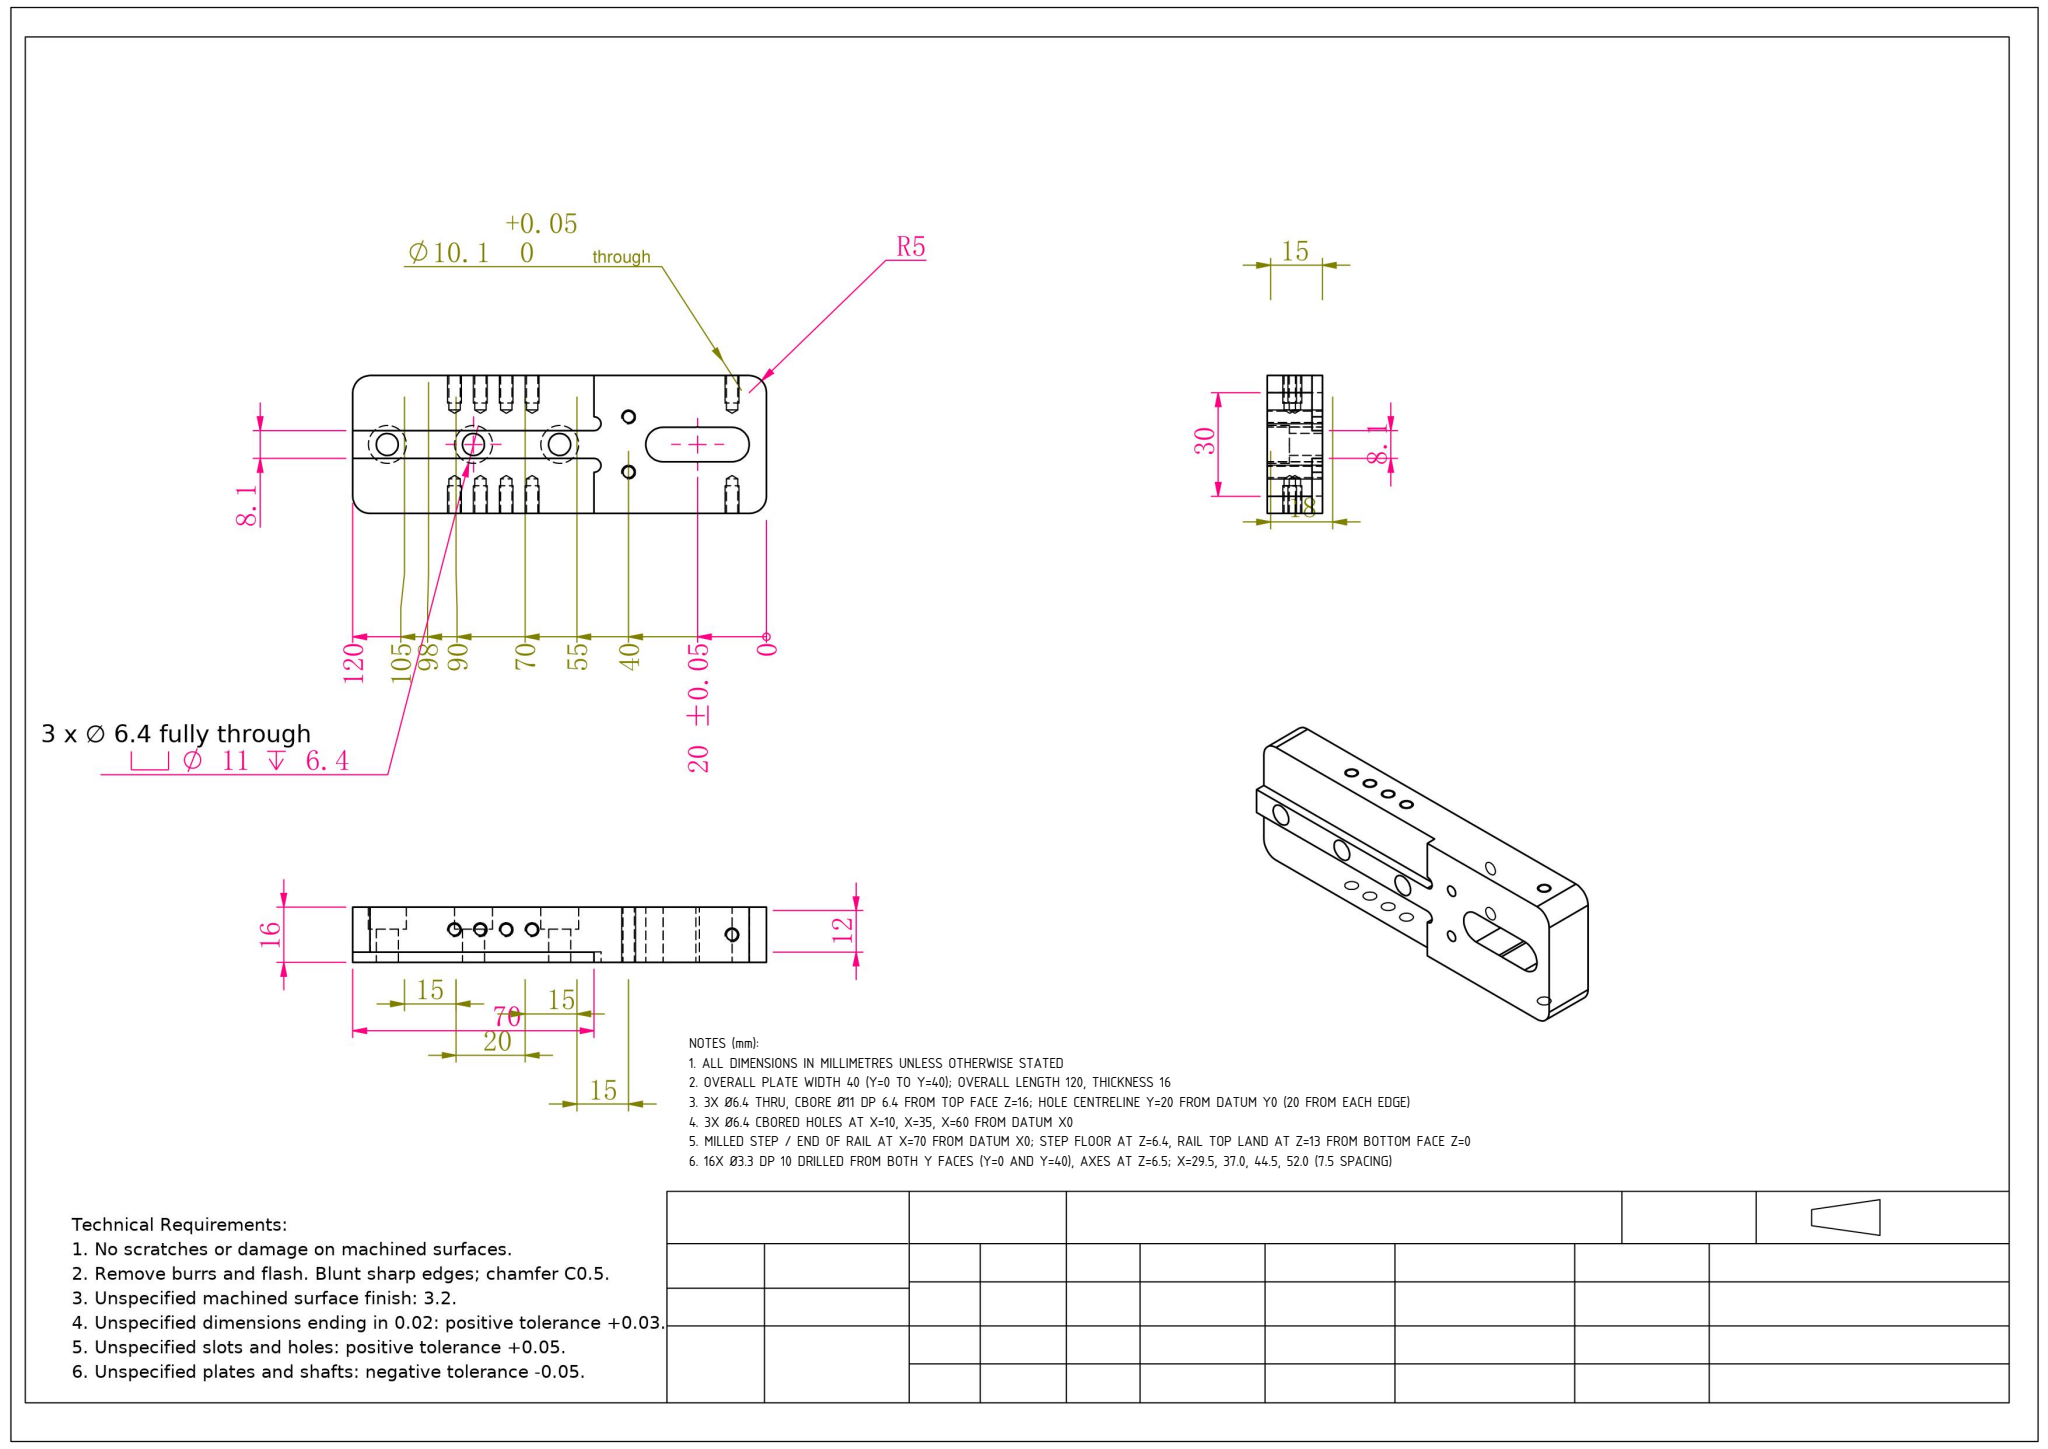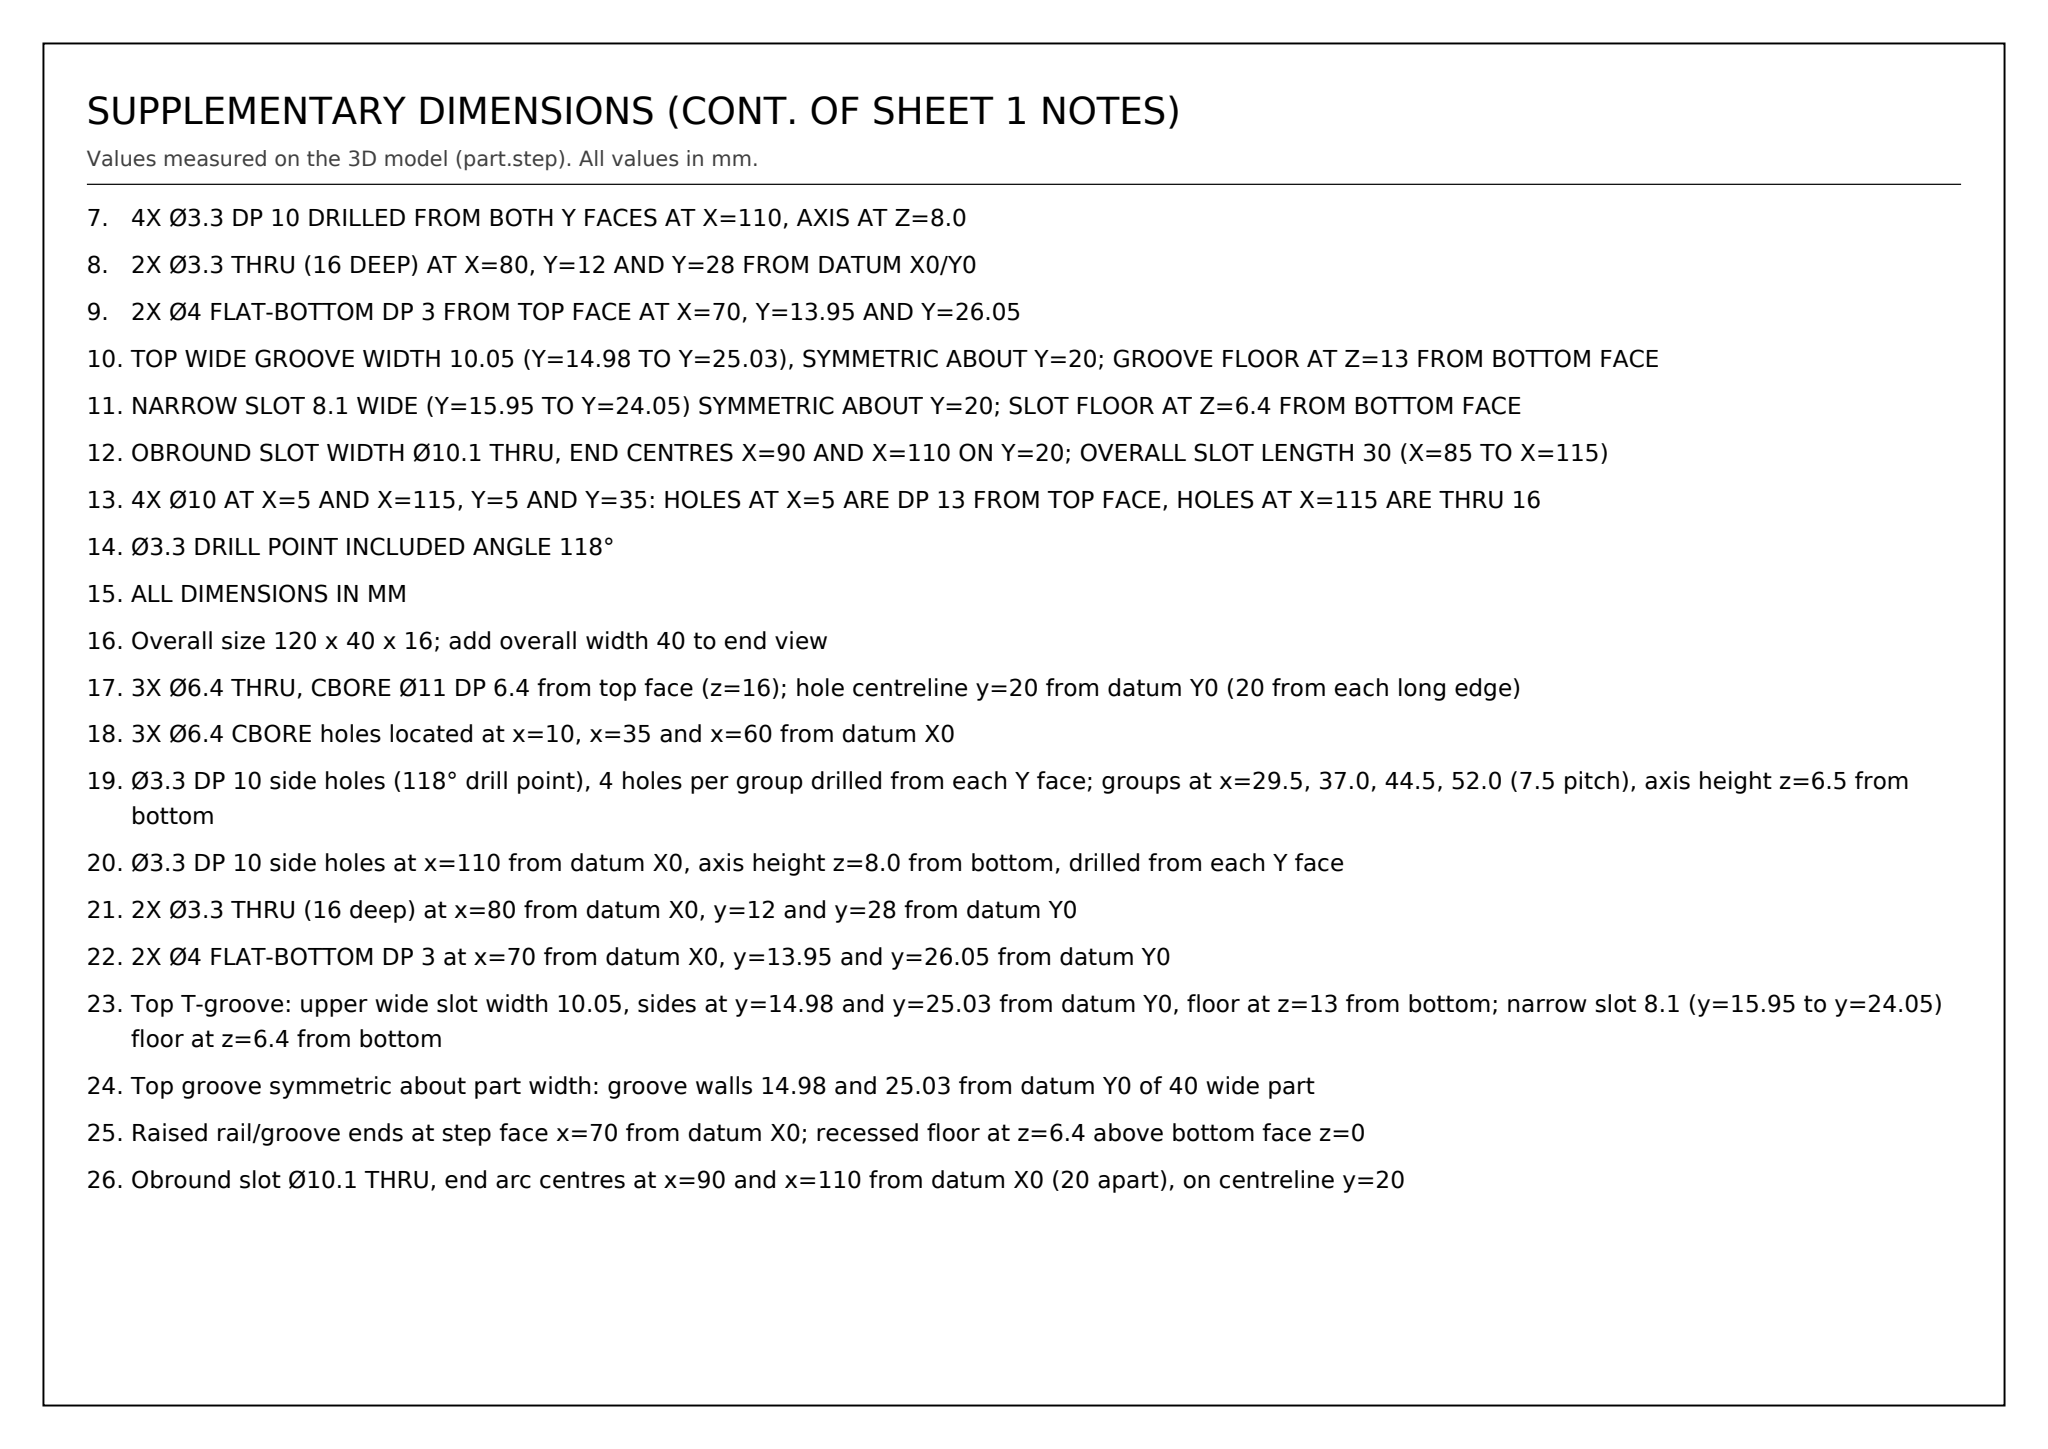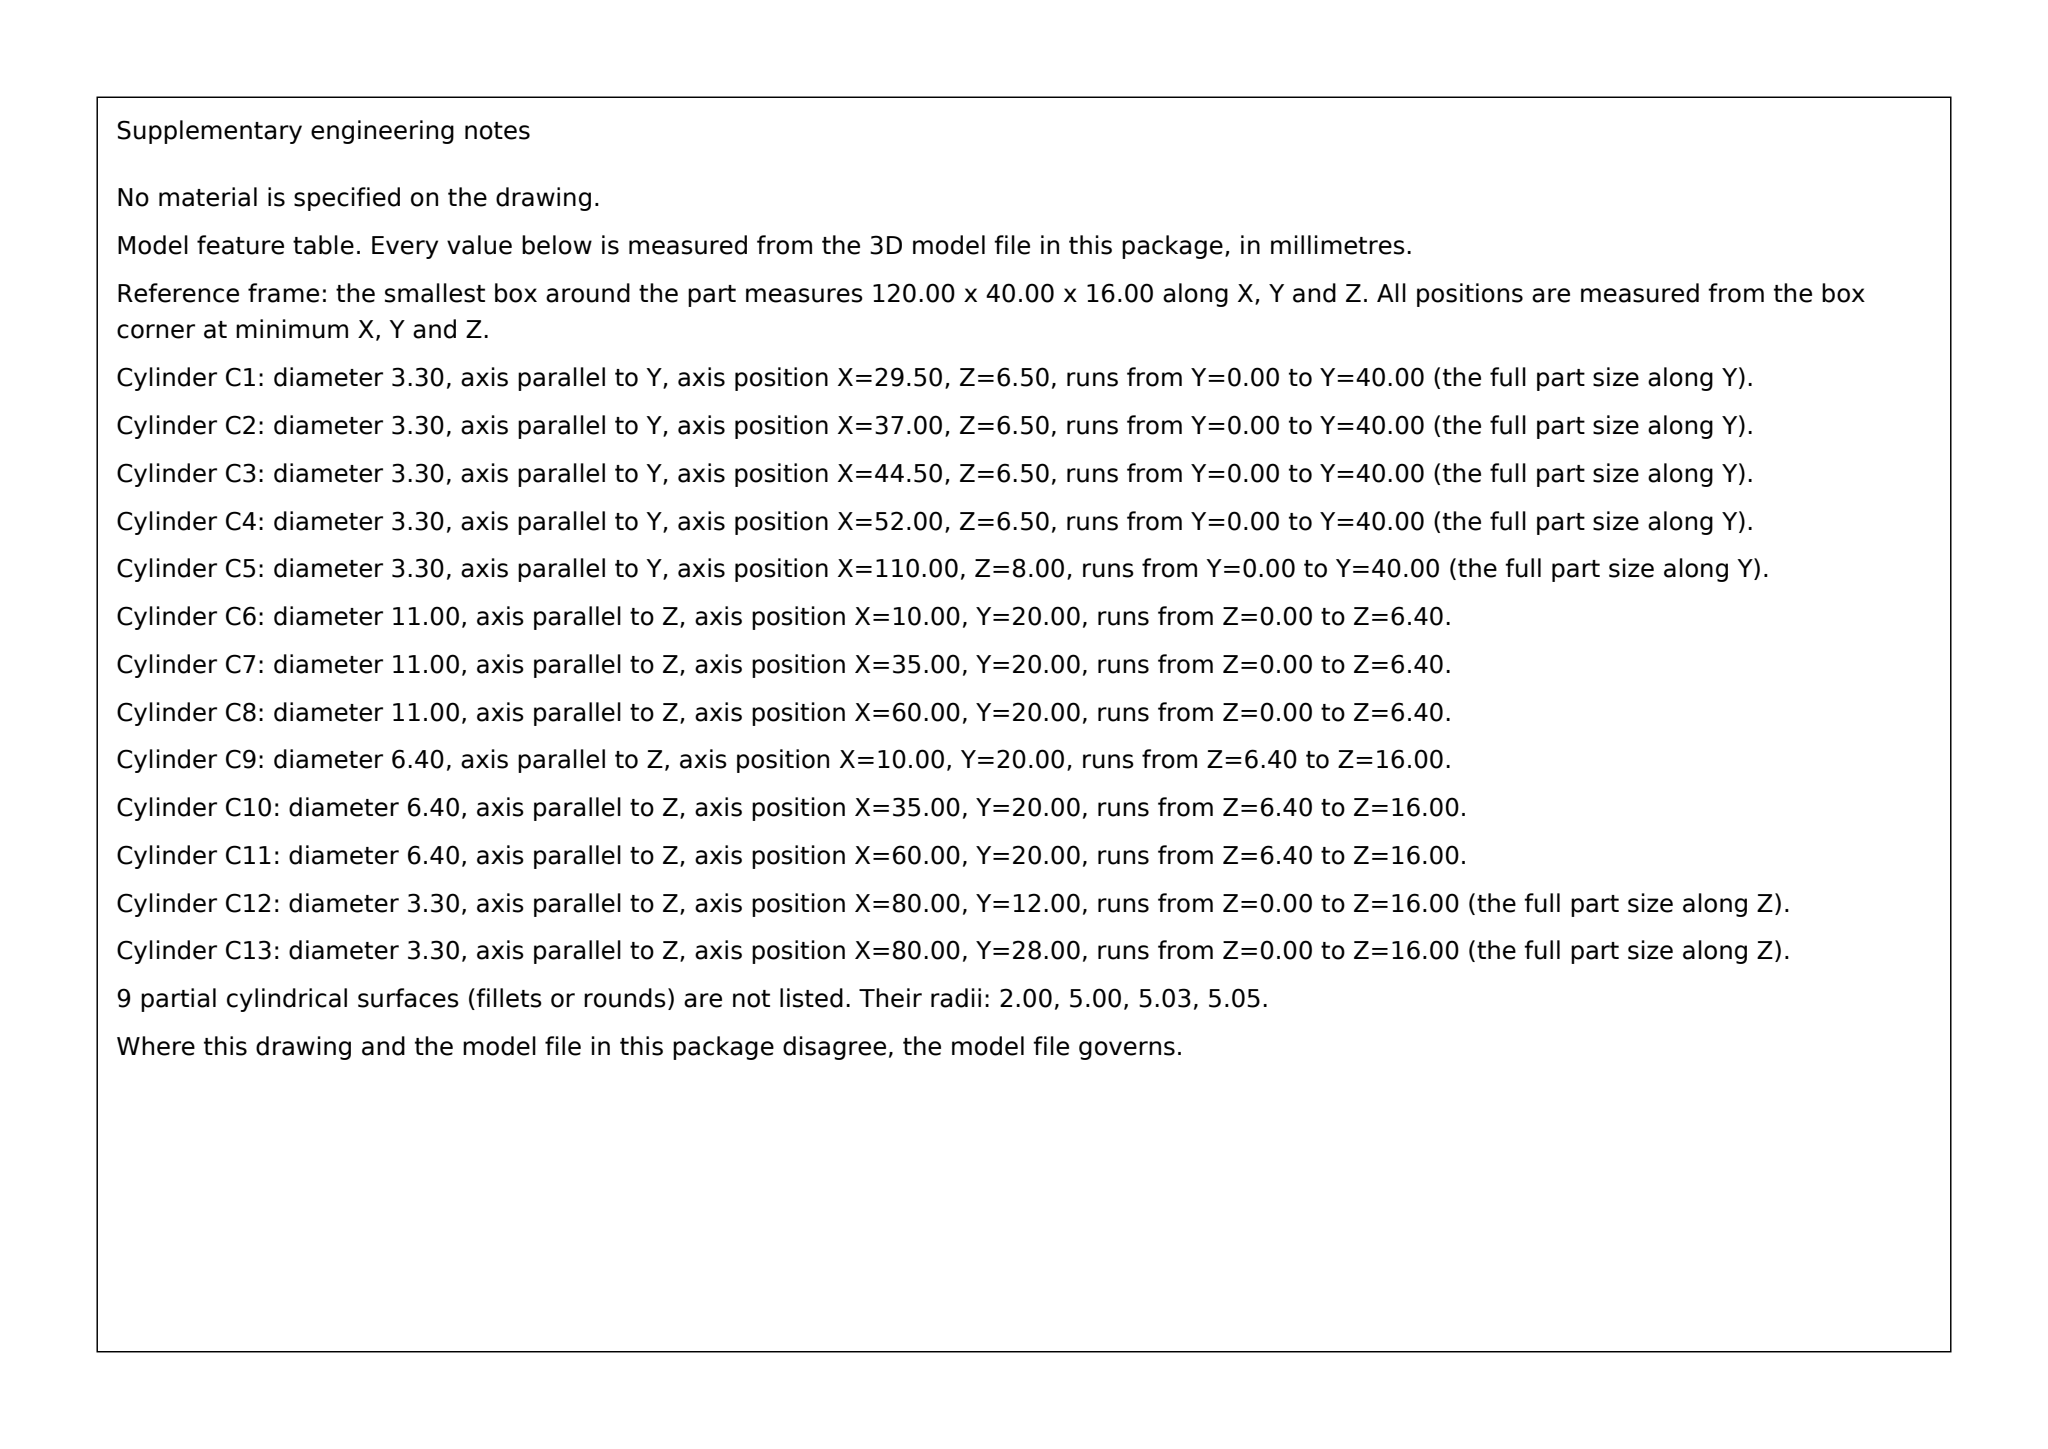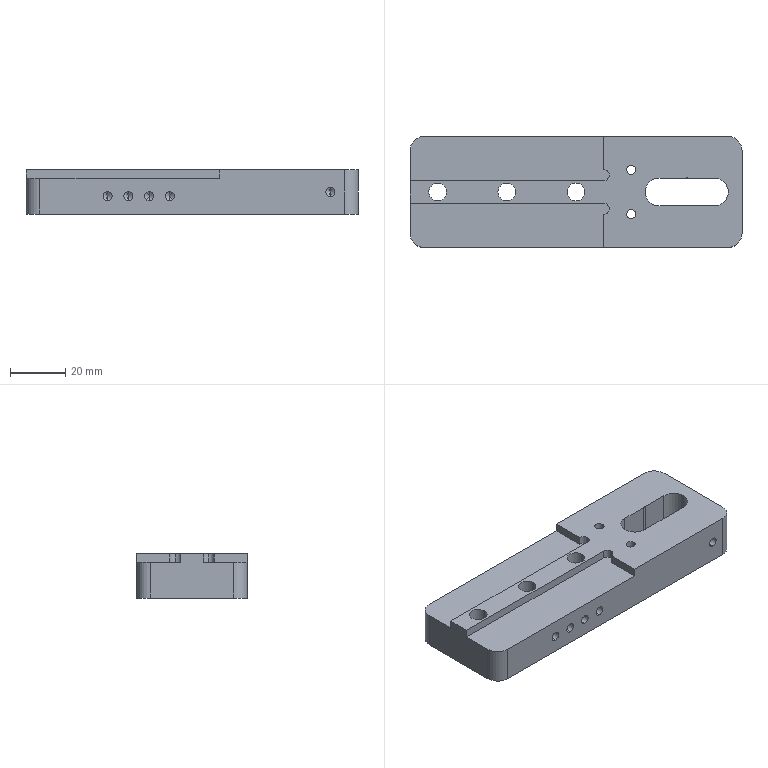Part | SolidWorks | mm | 1 solid | 88 faces | box 120 x 40 x 16 mm | volume 61358 mm3 | cylinder 49 | cone 20 | plane 19 | commonest cylinder face diameters 3.3 x24 11 x6 6.4 x6 4 x4 10 x4 10.05 x3 10.1 x2
Drawing notes:
ALL DIMENSIONS IN MILLIMETRES UNLESS OTHERWISE STATED | from the solid: STEP model units: mm (bbox_xyz 120.0 x 40.0 x 16.0)
OVERALL PLATE WIDTH 40 (Y=0 TO Y=40); OVERALL LENGTH 120, THICKNESS 16 | from the solid: bbox_xyz [120.0, 40.0, 16.0]
3X Ø6.4 THRU, CBORE Ø11 DP 6.4 FROM TOP FACE Z=16; HOLE CENTRELINE Y=20 FROM DATUM Y0 (20 FROM EACH EDGE) | from the solid: cylinders 6.4 z at y=20 len 9.6 and 11.0 z at y=20 len 6.4
3X Ø6.4 CBORED HOLES AT X=10, X=35, X=60 FROM DATUM X0 | from the solid: cylinders 6.4/11.0 z at pos x = 10.0, 35.0, 60.0
MILLED STEP / END OF RAIL AT X=70 FROM DATUM X0; STEP FLOOR AT Z=6.4, RAIL TOP LAND AT Z=13 FROM BOTTOM FACE Z=0 | from the solid: axis_planes x=70.0 (2), z=6.4 (3), z=13.0 (2)
16X Ø3.3 DP 10 DRILLED FROM BOTH Y FACES (Y=0 AND Y=40), AXES AT Z=6.5; X=29.5, 37.0, 44.5, 52.0 (7.5 SPACING) | from the solid: cylinders 3.3 axis y at [29.5/37.0/44.5/52.0, -, 6.5] length 10.0, count 4 each
4X Ø3.3 DP 10 DRILLED FROM BOTH Y FACES AT X=110, AXIS AT Z=8.0 | from the solid: cylinder 3.3 axis y at [110.0, -, 8.0] length 10.0 count 4
2X Ø3.3 THRU (16 DEEP) AT X=80, Y=12 AND Y=28 FROM DATUM X0/Y0 | from the solid: cylinders 3.3 axis z at [80.0, 12.0] and [80.0, 28.0] length 16.0
2X Ø4 FLAT-BOTTOM DP 3 FROM TOP FACE AT X=70, Y=13.95 AND Y=26.05 | from the solid: cylinders 4.0 axis z at [70.0, 13.95] and [70.0, 26.05] length 3.0
TOP WIDE GROOVE WIDTH 10.05 (Y=14.98 TO Y=25.03), SYMMETRIC ABOUT Y=20; GROOVE FLOOR AT Z=13 FROM BOTTOM FACE | from the solid: axis_planes y=14.98 (2) and y=25.03 (2); z=13.0 (2)
NARROW SLOT 8.1 WIDE (Y=15.95 TO Y=24.05) SYMMETRIC ABOUT Y=20; SLOT FLOOR AT Z=6.4 FROM BOTTOM FACE | from the solid: axis_planes y=15.95, y=24.05, z=6.4 (3)
OBROUND SLOT WIDTH Ø10.1 THRU, END CENTRES X=90 AND X=110 ON Y=20; OVERALL SLOT LENGTH 30 (X=85 TO X=115) | from the solid: cylinders 10.05 z at [90.0,20.0] and [110.0,20.0], 10.1 z at [100.0,20.0], all length 16.0 (thru)
4X Ø10 AT X=5 AND X=115, Y=5 AND Y=35: HOLES AT X=5 ARE DP 13 FROM TOP FACE, HOLES AT X=115 ARE THRU 16 | from the solid: cylinders 10.0 z at [5.0,5.0] and [5.0,35.0] length 13.0; [115.0,5.0] and [115.0,35.0] length 16.0
Ø3.3 DRILL POINT INCLUDED ANGLE 118° | from the solid: cones [118.0, ref_dia 3.3]
ALL DIMENSIONS IN MM | from the solid: STEP model facts stated in mm
Overall size 120 x 40 x 16; add overall width 40 to end view | from the solid: bbox_xyz [120.0, 40.0, 16.0]
3X Ø6.4 THRU, CBORE Ø11 DP 6.4 from top face (z=16); hole centreline y=20 from datum Y0 (20 from each long edge) | from the solid: cylinders 6.4 axis z pos y=20 len 9.6 and 11.0 axis z len 6.4
3X Ø6.4 CBORE holes located at x=10, x=35 and x=60 from datum X0 | from the solid: cylinders 6.4/11.0 axis z at x=10.0, 35.0, 60.0
Ø3.3 DP 10 side holes (118° drill point), 4 holes per group drilled from each Y face; groups at x=29.5, 37.0, 44.5, 52.0 (7.5 pitch), axis height z=6.5 from bottom | from the solid: cylinders [3.3,'y',[29.5/37.0/44.5/52.0,null,6.5],10.0,4]; cones [118.0, 3.3]
Ø3.3 DP 10 side holes at x=110 from datum X0, axis height z=8.0 from bottom, drilled from each Y face | from the solid: cylinders [3.3,'y',[110.0,null,8.0],10.0,4]
2X Ø3.3 THRU (16 deep) at x=80 from datum X0, y=12 and y=28 from datum Y0 | from the solid: cylinders [3.3,'z',[80.0,12.0],16.0] and [3.3,'z',[80.0,28.0],16.0]
2X Ø4 FLAT-BOTTOM DP 3 at x=70 from datum X0, y=13.95 and y=26.05 from datum Y0 | from the solid: cylinders [4.0,'z',[70.0,13.95],3.0] and [4.0,'z',[70.0,26.05],3.0]
Top T-groove: upper wide slot width 10.05, sides at y=14.98 and y=25.03 from datum Y0, floor at z=13 from bottom; narrow slot 8.1 (y=15.95 to y=24.05) floor at z=6.4 from bottom | from the solid: axis_planes y=14.98, y=25.03, y=15.95, y=24.05, z=13.0, z=6.4
Top groove symmetric about part width: groove walls 14.98 and 25.03 from datum Y0 of 40 wide part | from the solid: axis_planes y=14.98 / y=25.03 with bbox width 40.0
Raised rail/groove ends at step face x=70 from datum X0; recessed floor at z=6.4 above bottom face z=0 | from the solid: axis_planes x=70.0 (2) and z=6.4 (3), z=0.0
Obround slot Ø10.1 THRU, end arc centres at x=90 and x=110 from datum X0 (20 apart), on centreline y=20 | from the solid: cylinders [10.05,'z',[90.0,20.0],16.0], [10.05,'z',[110.0,20.0],16.0], [10.1,'z',[100.0,20.0],16.0]
build123d program:
from build123d import *

# Parameters (mm, degrees)
BOSS_EXTRUDE1_DEPTH                             = 12
BOSS_EXTRUDE1_DEPTH_BACK                        = 1
SKETCH1_W                                       = 120
SKETCH1_H                                       = 40
SKETCH3_W                                       = 70
SKETCH3_H                                       = 8.1
BOSS_EXTRUDE3_DEPTH                             = 3
M6_HEX_SOCKET_HEAD_CAP_SCREW_CBORE1_D           = 6.4
M6_HEX_SOCKET_HEAD_CAP_SCREW_CBORE1_CBORE_D     = 11
M6_HEX_SOCKET_HEAD_CAP_SCREW_CBORE1_CBORE_DEPTH = 6.4
SKETCH9_W                                       = 50
SKETCH9_H                                       = 40
BOSS_EXTRUDE4_DEPTH                             = 3
SKETCH4_R                                       = 5.05
CUT_EXTRUDE1_DEPTH                              = 123.703
SKETCH10_R                                      = 2
CUT_EXTRUDE2_DEPTH                              = 3
FILLET1_R                                       = 5
M4_TAPPED_HOLE2_AT_2_COUNT                      = 2
M4_TAPPED_HOLE2_AT_2_PITCH                      = 15
M4_TAPPED_HOLE2_AT_3_COUNT                      = 2
M4_TAPPED_HOLE2_AT_3_PITCH                      = 7.5
M4_TAPPED_HOLE2_AT_4_COUNT                      = 2
M4_TAPPED_HOLE2_AT_4_PITCH                      = 7.5
CUT_EXTRUDE3_DEPTH                              = 123.703
M4_TAPPED_HOLE3_D                               = 3.3


with BuildPart() as part:
    # Sketch1 → Boss-Extrude1 (new, two sides: drawn at the far end of the back side and taken through both)
    with BuildSketch(Plane.XY.offset(-BOSS_EXTRUDE1_DEPTH_BACK)):
        with Locations((60, 0)):
            Rectangle(SKETCH1_W, SKETCH1_H)
    extrude(amount=BOSS_EXTRUDE1_DEPTH + BOSS_EXTRUDE1_DEPTH_BACK)

    # Sketch3 → Boss-Extrude3 (add)
    with BuildSketch(Plane.XY.offset(12)):
        with Locations((35, 0)):
            Rectangle(SKETCH3_W, SKETCH3_H)
    extrude(amount=BOSS_EXTRUDE3_DEPTH)

    # M6 Hex Socket Head Cap Screw CBORE1 (through all)
    with Locations(Plane(origin=(0, 0, -1), x_dir=(-1, 0, 0), z_dir=(0, 0, -1))):
        with Locations((-10, 0), (-35, 0), (-60, 0)):
            CounterBoreHole(M6_HEX_SOCKET_HEAD_CAP_SCREW_CBORE1_D / 2, M6_HEX_SOCKET_HEAD_CAP_SCREW_CBORE1_CBORE_D / 2, M6_HEX_SOCKET_HEAD_CAP_SCREW_CBORE1_CBORE_DEPTH)

    # Sketch9 → Boss-Extrude4 (add)
    with BuildSketch(Plane.XY.offset(12)):
        with Locations((95, 0)):
            Rectangle(SKETCH9_W, SKETCH9_H)
    extrude(amount=BOSS_EXTRUDE4_DEPTH)

    # Sketch4 → Cut-Extrude1 (cut, through all)
    with BuildSketch(Plane.XY.offset(-1)):
        with Locations((100, 0)):
            Circle(SKETCH4_R)
    extrude(amount=CUT_EXTRUDE1_DEPTH, mode=Mode.SUBTRACT)

    # Sketch10 → Cut-Extrude2 (cut)
    with BuildSketch(Plane.XY.offset(15)):
        with Locations((70, 6.05)):
            Circle(SKETCH10_R)
        with Locations((70, -6.05)):
            Circle(SKETCH10_R)
    extrude(amount=-CUT_EXTRUDE2_DEPTH, mode=Mode.SUBTRACT)

    # Fillet1
    fillet1_edges = [part.edges().sort_by_distance(p)[0] for p in [
        (0, 20, 5.5),
        (120, 20, 7),
        (120, -20, 7),
        (0, -20, 5.5),
    ]]
    fillet(fillet1_edges, radius=FILLET1_R)

    # Sketch14 → M4 Tapped Hole1 (revolve, cut)
    with BuildSketch(Plane(origin=(110, 20, 7), x_dir=(0, 0, 1), z_dir=(1, 0, 0))):
        Polygon((0, 0), (0, 10.991), (1.65, 10), (1.65, 0), align=None)
    m4_tapped_hole1 = revolve(axis=Axis((110, 26.35, 7), (0, -1, 0)), mode=Mode.SUBTRACT)

    # Sketch16 → M4 Tapped Hole2 (revolve, cut)
    with BuildSketch(Plane(origin=(37, 20, 5.5), x_dir=(0, 0, 1), z_dir=(1, 0, 0))):
        Polygon((0, 0), (0, 10.991), (1.65, 10), (1.65, 0), align=None)
    m4_tapped_hole2 = revolve(axis=Axis((37, 26.35, 5.5), (0, -1, 0)), mode=Mode.SUBTRACT)

    # M4 Tapped Hole2 at 2: M4 Tapped Hole2 ×2
    with Locations(*[(i * M4_TAPPED_HOLE2_AT_2_PITCH, 0, 0) for i in range(1, M4_TAPPED_HOLE2_AT_2_COUNT)]):
        add(m4_tapped_hole2, mode=Mode.SUBTRACT)

    # M4 Tapped Hole2 at 3: M4 Tapped Hole2 ×2
    with Locations(*[(i * M4_TAPPED_HOLE2_AT_3_PITCH, 0, 0) for i in range(1, M4_TAPPED_HOLE2_AT_3_COUNT)]):
        add(m4_tapped_hole2, mode=Mode.SUBTRACT)

    # M4 Tapped Hole2 at 4: M4 Tapped Hole2 ×2
    with Locations(*[(-i * M4_TAPPED_HOLE2_AT_4_PITCH, 0, 0) for i in range(1, M4_TAPPED_HOLE2_AT_4_COUNT)]):
        add(m4_tapped_hole2, mode=Mode.SUBTRACT)

    # Mirror1: M4 Tapped Hole1, M4 Tapped Hole2 across plane
    add(m4_tapped_hole1.mirror(Plane.ZX), mode=Mode.SUBTRACT)
    add(m4_tapped_hole2.mirror(Plane.ZX), mode=Mode.SUBTRACT)

    # Mirror1 copy 1 sketch → Mirror1 copy 1 (revolve, cut)
    with BuildSketch(Plane(origin=(52, -20, 5.5), x_dir=(0, 0, 1), z_dir=(1, 0, 0))):
        Polygon((0, 0), (0, -10.991), (1.65, -10), (1.65, 0), align=None)
    revolve(axis=Axis((52, -26.35, 5.5), (0, -1, 0)), mode=Mode.SUBTRACT)

    # Mirror1 copy 2 sketch → Mirror1 copy 2 (revolve, cut)
    with BuildSketch(Plane(origin=(44.5, -20, 5.5), x_dir=(0, 0, 1), z_dir=(1, 0, 0))):
        Polygon((0, 0), (0, -10.991), (1.65, -10), (1.65, 0), align=None)
    revolve(axis=Axis((44.5, -26.35, 5.5), (0, -1, 0)), mode=Mode.SUBTRACT)

    # Mirror1 copy 3 sketch → Mirror1 copy 3 (revolve, cut)
    with BuildSketch(Plane(origin=(29.5, -20, 5.5), x_dir=(0, 0, 1), z_dir=(1, 0, 0))):
        Polygon((0, 0), (0, -10.991), (1.65, -10), (1.65, 0), align=None)
    revolve(axis=Axis((29.5, -26.35, 5.5), (0, -1, 0)), mode=Mode.SUBTRACT)

    # Sketch17 → Cut-Extrude3 (cut, through all)
    with BuildSketch(Plane.XY.offset(15)):
        with BuildLine():
            Line((90, 5.025), (110, 5.025))
            ThreePointArc((110, 5.025), (115.025, 0), (110, -5.025))
            Line((110, -5.025), (90, -5.025))
            ThreePointArc((90, -5.025), (84.975, 0), (90, 5.025))
        make_face()
    extrude(amount=-CUT_EXTRUDE3_DEPTH, mode=Mode.SUBTRACT)

    # M4 Tapped Hole3 (through all)
    with Locations(Plane(origin=(0, 0, -1), x_dir=(-1, 0, 0), z_dir=(0, 0, -1))):
        with Locations((-80, 8), (-80, -8)):
            Hole(M4_TAPPED_HOLE3_D / 2)


solid = part.part